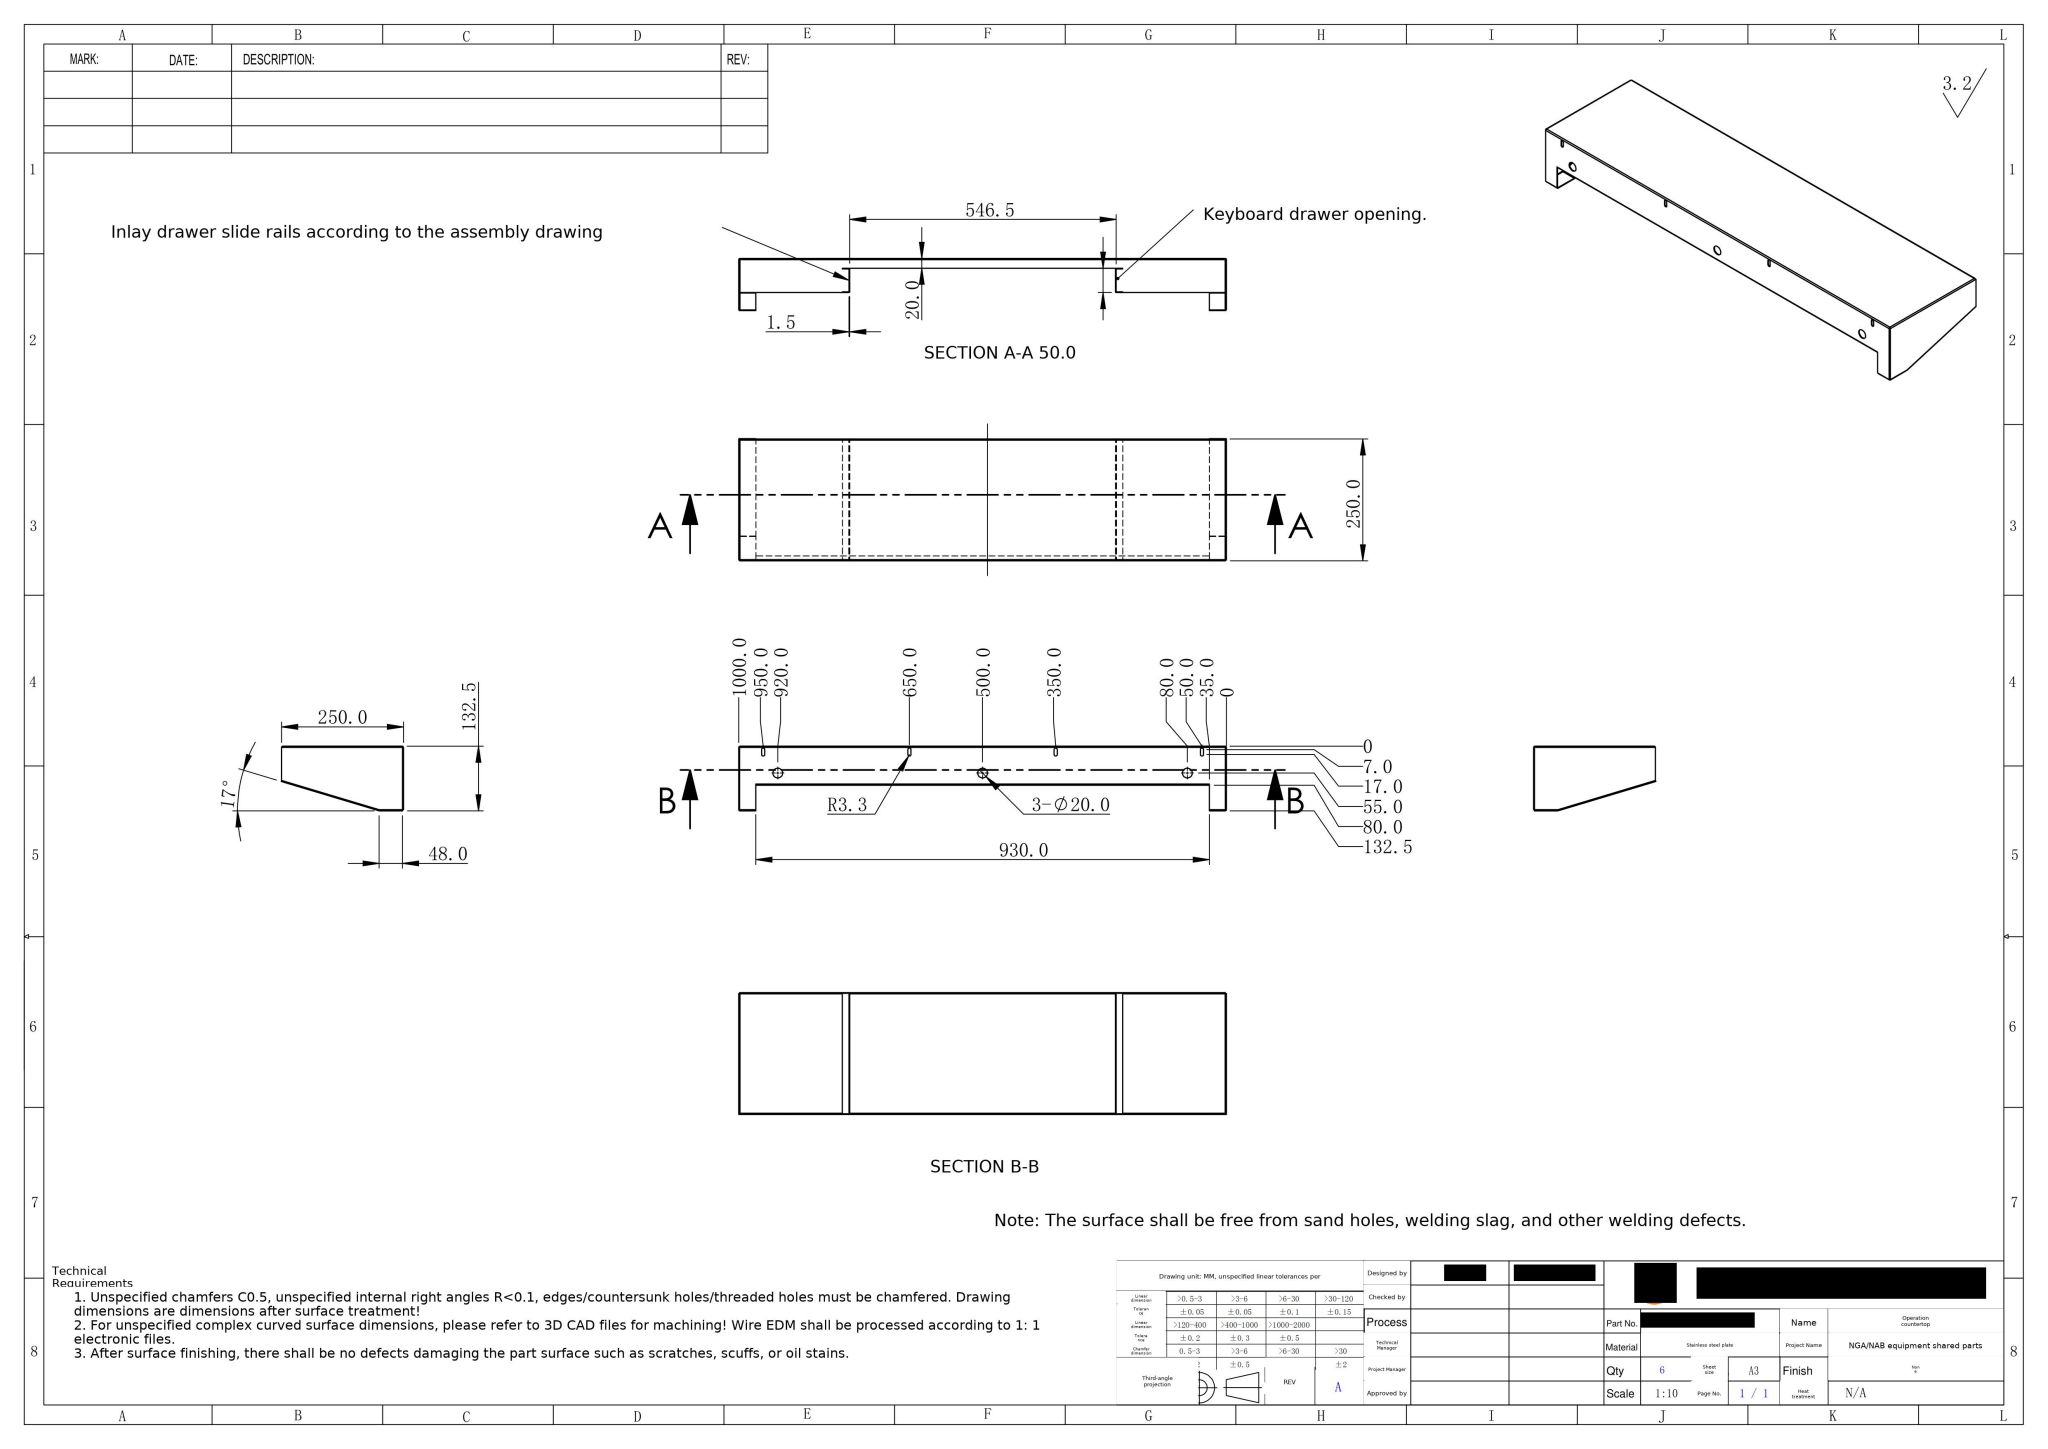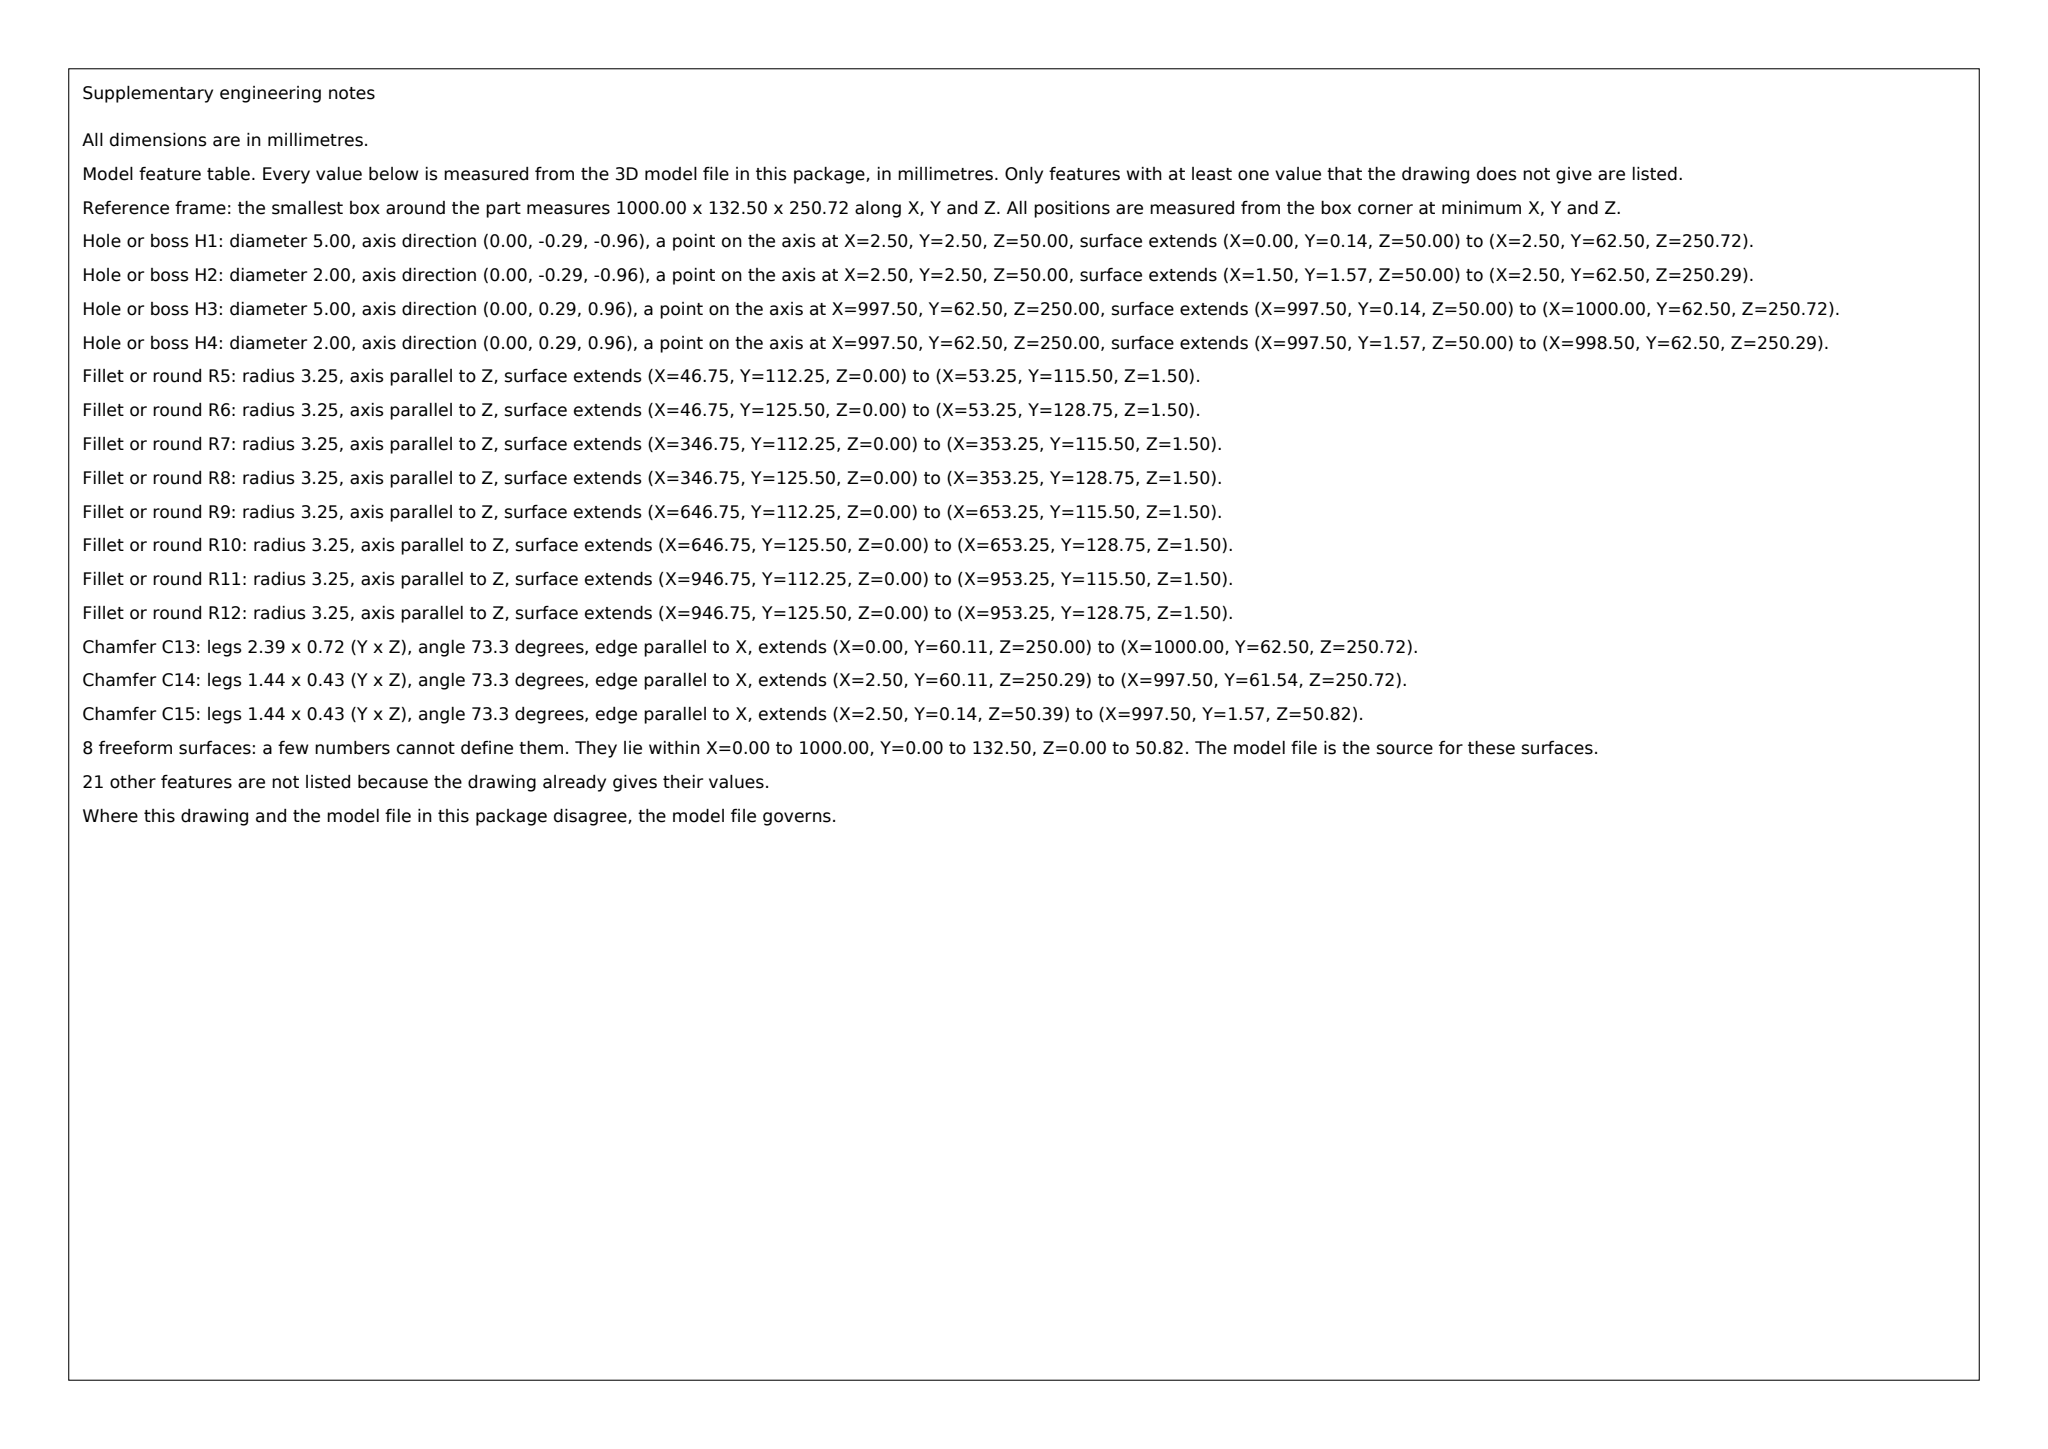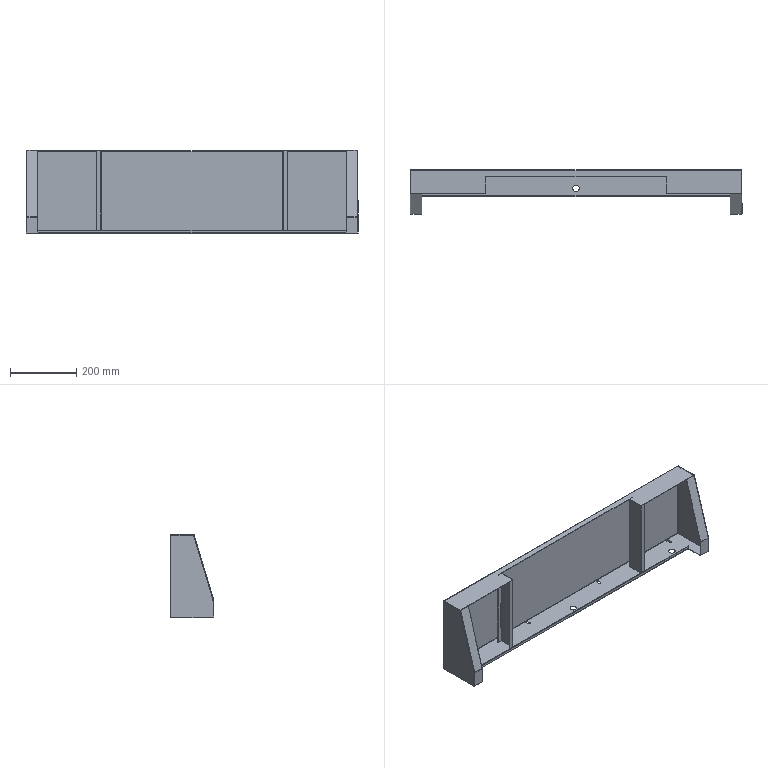Part | SolidWorks | mm | material Stainless steel plate | 1 solid | 129 faces | box 1000 x 132.5 x 250.72 mm | volume 725633 mm3 | plane 84 | cylinder 37 | spline 8 | commonest cylinder face diameters 5 x9 2 x9 6.5 x8 20 x6 4 x5